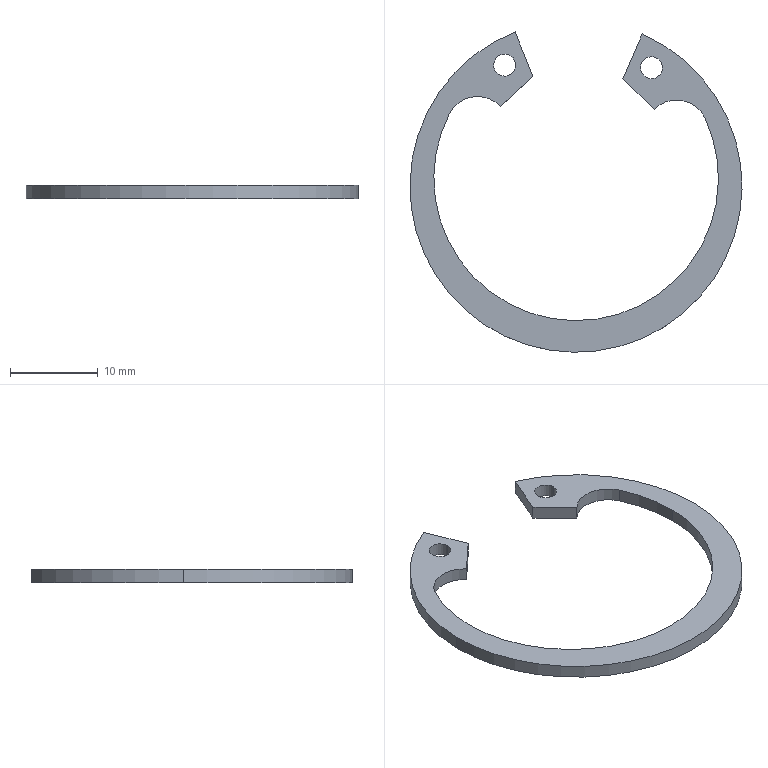Component | SolidWorks | HopperAssembly-1_20211103-210426-70669.STEP-1_-_-_-1.STEP-1_GB893_2-86_B_35.STEP-1 | 1 solid | 18 faces | box 37.8 x 36.49 x 1.5 mm | volume 478 mm3 | cylinder 12 | plane 6 | commonest cylinder face diameters 2.5 x4 32.4 x3 37.8 x3 7.2 x2
STEP:
#1=CARTESIAN_POINT('',(-115.828,33.727,-14.858));
#2=VERTEX_POINT('',#1);
#3=CARTESIAN_POINT('',(-115.927,33.729,-14.858));
#4=VERTEX_POINT('',#3);
#5=CARTESIAN_POINT('',(-115.877,33.728,-14.858));
#6=DIRECTION('',(-0.,-0.,1.));
#7=DIRECTION('',(-0.9998,0.01747,0.));
#8=AXIS2_PLACEMENT_3D('',#5,#6,#7);
#9=CIRCLE('',#8,0.04921);
#10=EDGE_CURVE('',#2,#4,#9,.T.);
#11=ORIENTED_EDGE('',*,*,#10,.T.);
#12=CARTESIAN_POINT('',(-115.877,33.728,-14.858));
#13=DIRECTION('',(-0.,-0.,1.));
#14=DIRECTION('',(-0.9998,0.01747,0.));
#15=AXIS2_PLACEMENT_3D('',#12,#13,#14);
#16=CIRCLE('',#15,0.04921);
#17=EDGE_CURVE('',#4,#2,#16,.T.);
#18=ORIENTED_EDGE('',*,*,#17,.T.);
#19=EDGE_LOOP('',(#11,#18));
#20=FACE_BOUND('',#19,.T.);
#21=CARTESIAN_POINT('',(-116.486,33.738,-14.858));
#22=VERTEX_POINT('',#21);
#23=CARTESIAN_POINT('',(-116.585,33.74,-14.858));
#24=VERTEX_POINT('',#23);
#25=CARTESIAN_POINT('',(-116.535,33.739,-14.858));
#26=DIRECTION('',(-0.,-0.,1.));
#27=DIRECTION('',(0.9998,-0.01747,0.));
#28=AXIS2_PLACEMENT_3D('',#25,#26,#27);
#29=CIRCLE('',#28,0.04921);
#30=EDGE_CURVE('',#22,#24,#29,.T.);
#31=ORIENTED_EDGE('',*,*,#30,.T.);
#32=CARTESIAN_POINT('',(-116.535,33.739,-14.858));
#33=DIRECTION('',(-0.,-0.,1.));
#34=DIRECTION('',(0.9998,-0.01747,0.));
#35=AXIS2_PLACEMENT_3D('',#32,#33,#34);
#36=CIRCLE('',#35,0.04921);
#37=EDGE_CURVE('',#24,#22,#36,.T.);
#38=ORIENTED_EDGE('',*,*,#37,.T.);
#39=EDGE_LOOP('',(#31,#38));
#40=FACE_BOUND('',#39,.T.);
#41=CARTESIAN_POINT('',(-116.489,33.889,-14.858));
#42=VERTEX_POINT('',#41);
#43=CARTESIAN_POINT('',(-116.96,33.209,-14.858));
#44=VERTEX_POINT('',#43);
#45=CARTESIAN_POINT('',(-116.216,33.196,-14.858));
#46=DIRECTION('',(-0.,-0.,1.));
#47=DIRECTION('',(-0.9998,0.01747,0.));
#48=AXIS2_PLACEMENT_3D('',#45,#46,#47);
#49=CIRCLE('',#48,0.7441);
#50=EDGE_CURVE('',#42,#44,#49,.T.);
#51=ORIENTED_EDGE('',*,*,#50,.F.);
#52=CARTESIAN_POINT('',(-116.409,33.687,-14.858));
#53=VERTEX_POINT('',#52);
#54=CARTESIAN_POINT('',(-116.409,33.687,-14.858));
#55=DIRECTION('',(-0.3665,0.9304,0.));
#56=VECTOR('',#55,39.37);
#57=LINE('',#54,#56);
#58=EDGE_CURVE('',#53,#42,#57,.T.);
#59=ORIENTED_EDGE('',*,*,#58,.F.);
#60=CARTESIAN_POINT('',(-116.553,33.553,-14.858));
#61=VERTEX_POINT('',#60);
#62=CARTESIAN_POINT('',(-116.553,33.553,-14.858));
#63=DIRECTION('',(0.7328,0.6804,0.));
#64=VECTOR('',#63,39.37);
#65=LINE('',#62,#64);
#66=EDGE_CURVE('',#61,#53,#65,.T.);
#67=ORIENTED_EDGE('',*,*,#66,.F.);
#68=CARTESIAN_POINT('',(-116.784,33.521,-14.858));
#69=VERTEX_POINT('',#68);
#70=CARTESIAN_POINT('',(-116.657,33.457,-14.858));
#71=DIRECTION('',(0.,0.,-1.));
#72=DIRECTION('',(0.9998,-0.01747,0.));
#73=AXIS2_PLACEMENT_3D('',#70,#71,#72);
#74=CIRCLE('',#73,0.1417);
#75=EDGE_CURVE('',#69,#61,#74,.T.);
#76=ORIENTED_EDGE('',*,*,#75,.F.);
#77=CARTESIAN_POINT('',(-116.853,33.243,-14.858));
#78=VERTEX_POINT('',#77);
#79=CARTESIAN_POINT('',(-116.215,33.232,-14.858));
#80=DIRECTION('',(0.,0.,-1.));
#81=DIRECTION('',(-0.9998,0.01747,0.));
#82=AXIS2_PLACEMENT_3D('',#79,#80,#81);
#83=CIRCLE('',#82,0.6378);
#84=EDGE_CURVE('',#78,#69,#83,.T.);
#85=ORIENTED_EDGE('',*,*,#84,.F.);
#86=CARTESIAN_POINT('',(-115.578,33.221,-14.858));
#87=VERTEX_POINT('',#86);
#88=CARTESIAN_POINT('',(-116.215,33.232,-14.858));
#89=DIRECTION('',(0.,0.,-1.));
#90=DIRECTION('',(-0.9998,0.01747,0.));
#91=AXIS2_PLACEMENT_3D('',#88,#89,#90);
#92=CIRCLE('',#91,0.6378);
#93=EDGE_CURVE('',#87,#78,#92,.T.);
#94=ORIENTED_EDGE('',*,*,#93,.F.);
#95=CARTESIAN_POINT('',(-115.637,33.501,-14.858));
#96=VERTEX_POINT('',#95);
#97=CARTESIAN_POINT('',(-116.215,33.232,-14.858));
#98=DIRECTION('',(0.,0.,-1.));
#99=DIRECTION('',(-0.9998,0.01747,0.));
#100=AXIS2_PLACEMENT_3D('',#97,#98,#99);
#101=CIRCLE('',#100,0.6378);
#102=EDGE_CURVE('',#96,#87,#101,.T.);
#103=ORIENTED_EDGE('',*,*,#102,.F.);
#104=CARTESIAN_POINT('',(-115.866,33.541,-14.858));
#105=VERTEX_POINT('',#104);
#106=CARTESIAN_POINT('',(-115.766,33.441,-14.858));
#107=DIRECTION('',(0.,0.,-1.));
#108=DIRECTION('',(-0.9998,0.01747,0.));
#109=AXIS2_PLACEMENT_3D('',#106,#107,#108);
#110=CIRCLE('',#109,0.1417);
#111=EDGE_CURVE('',#105,#96,#110,.T.);
#112=ORIENTED_EDGE('',*,*,#111,.F.);
#113=CARTESIAN_POINT('',(-116.005,33.68,-14.858));
#114=VERTEX_POINT('',#113);
#115=CARTESIAN_POINT('',(-115.866,33.541,-14.858));
#116=DIRECTION('',(0.7086,-0.7056,-0.));
#117=VECTOR('',#116,39.37);
#118=LINE('',#115,#117);
#119=EDGE_CURVE('',#114,#105,#118,.T.);
#120=ORIENTED_EDGE('',*,*,#119,.F.);
#121=CARTESIAN_POINT('',(-115.919,33.879,-14.858));
#122=VERTEX_POINT('',#121);
#123=CARTESIAN_POINT('',(-116.005,33.68,-14.858));
#124=DIRECTION('',(-0.3988,-0.9171,-0.));
#125=VECTOR('',#124,39.37);
#126=LINE('',#123,#125);
#127=EDGE_CURVE('',#122,#114,#126,.T.);
#128=ORIENTED_EDGE('',*,*,#127,.F.);
#129=CARTESIAN_POINT('',(-115.472,33.183,-14.858));
#130=VERTEX_POINT('',#129);
#131=CARTESIAN_POINT('',(-116.216,33.196,-14.858));
#132=DIRECTION('',(-0.,-0.,1.));
#133=DIRECTION('',(-0.9998,0.01747,0.));
#134=AXIS2_PLACEMENT_3D('',#131,#132,#133);
#135=CIRCLE('',#134,0.7441);
#136=EDGE_CURVE('',#130,#122,#135,.T.);
#137=ORIENTED_EDGE('',*,*,#136,.F.);
#138=CARTESIAN_POINT('',(-116.216,33.196,-14.858));
#139=DIRECTION('',(-0.,-0.,1.));
#140=DIRECTION('',(-0.9998,0.01747,0.));
#141=AXIS2_PLACEMENT_3D('',#138,#139,#140);
#142=CIRCLE('',#141,0.7441);
#143=EDGE_CURVE('',#44,#130,#142,.T.);
#144=ORIENTED_EDGE('',*,*,#143,.F.);
#145=EDGE_LOOP('',(#51,#59,#67,#76,#85,#94,#103,#112,#120,#128,#137,#144));
#146=FACE_OUTER_BOUND('',#145,.T.);
#147=CARTESIAN_POINT('',(-116.216,33.196,-14.858));
#148=DIRECTION('',(-0.,-0.,1.));
#149=DIRECTION('',(-0.9998,0.01747,-0.));
#150=AXIS2_PLACEMENT_3D('',#147,#148,#149);
#151=PLANE('',#150);
#152=ADVANCED_FACE('',(#20,#40,#146),#151,.F.);
#153=CARTESIAN_POINT('',(-116.585,33.74,-14.799));
#154=VERTEX_POINT('',#153);
#155=CARTESIAN_POINT('',(-116.585,33.74,-14.799));
#156=DIRECTION('',(0.,0.,-1.));
#157=VECTOR('',#156,39.37);
#158=LINE('',#155,#157);
#159=EDGE_CURVE('',#154,#24,#158,.T.);
#160=ORIENTED_EDGE('',*,*,#159,.F.);
#161=CARTESIAN_POINT('',(-116.486,33.738,-14.799));
#162=VERTEX_POINT('',#161);
#163=CARTESIAN_POINT('',(-116.535,33.739,-14.799));
#164=DIRECTION('',(-0.,-0.,1.));
#165=DIRECTION('',(0.9998,-0.01747,0.));
#166=AXIS2_PLACEMENT_3D('',#163,#164,#165);
#167=CIRCLE('',#166,0.04921);
#168=EDGE_CURVE('',#154,#162,#167,.T.);
#169=ORIENTED_EDGE('',*,*,#168,.T.);
#170=CARTESIAN_POINT('',(-116.486,33.738,-14.799));
#171=DIRECTION('',(0.,0.,-1.));
#172=VECTOR('',#171,39.37);
#173=LINE('',#170,#172);
#174=EDGE_CURVE('',#162,#22,#173,.T.);
#175=ORIENTED_EDGE('',*,*,#174,.T.);
#176=ORIENTED_EDGE('',*,*,#37,.F.);
#177=EDGE_LOOP('',(#160,#169,#175,#176));
#178=FACE_OUTER_BOUND('',#177,.T.);
#179=CARTESIAN_POINT('',(-116.535,33.739,-14.799));
#180=DIRECTION('',(0.,0.,-1.));
#181=DIRECTION('',(0.9998,-0.01747,0.));
#182=AXIS2_PLACEMENT_3D('',#179,#180,#181);
#183=CYLINDRICAL_SURFACE('',#182,0.04921);
#184=ADVANCED_FACE('',(#178),#183,.F.);
#185=CARTESIAN_POINT('',(-115.927,33.729,-14.799));
#186=VERTEX_POINT('',#185);
#187=CARTESIAN_POINT('',(-115.927,33.729,-14.799));
#188=DIRECTION('',(0.,0.,-1.));
#189=VECTOR('',#188,39.37);
#190=LINE('',#187,#189);
#191=EDGE_CURVE('',#186,#4,#190,.T.);
#192=ORIENTED_EDGE('',*,*,#191,.F.);
#193=CARTESIAN_POINT('',(-115.828,33.727,-14.799));
#194=VERTEX_POINT('',#193);
#195=CARTESIAN_POINT('',(-115.877,33.728,-14.799));
#196=DIRECTION('',(-0.,-0.,1.));
#197=DIRECTION('',(-0.9998,0.01747,0.));
#198=AXIS2_PLACEMENT_3D('',#195,#196,#197);
#199=CIRCLE('',#198,0.04921);
#200=EDGE_CURVE('',#186,#194,#199,.T.);
#201=ORIENTED_EDGE('',*,*,#200,.T.);
#202=CARTESIAN_POINT('',(-115.828,33.727,-14.799));
#203=DIRECTION('',(0.,0.,-1.));
#204=VECTOR('',#203,39.37);
#205=LINE('',#202,#204);
#206=EDGE_CURVE('',#194,#2,#205,.T.);
#207=ORIENTED_EDGE('',*,*,#206,.T.);
#208=ORIENTED_EDGE('',*,*,#17,.F.);
#209=EDGE_LOOP('',(#192,#201,#207,#208));
#210=FACE_OUTER_BOUND('',#209,.T.);
#211=CARTESIAN_POINT('',(-115.877,33.728,-14.799));
#212=DIRECTION('',(0.,0.,-1.));
#213=DIRECTION('',(0.9998,-0.01747,0.));
#214=AXIS2_PLACEMENT_3D('',#211,#212,#213);
#215=CYLINDRICAL_SURFACE('',#214,0.04921);
#216=ADVANCED_FACE('',(#210),#215,.F.);
#217=CARTESIAN_POINT('',(-116.409,33.687,-14.799));
#218=VERTEX_POINT('',#217);
#219=CARTESIAN_POINT('',(-116.409,33.687,-14.799));
#220=DIRECTION('',(0.,0.,-1.));
#221=VECTOR('',#220,39.37);
#222=LINE('',#219,#221);
#223=EDGE_CURVE('',#218,#53,#222,.T.);
#224=ORIENTED_EDGE('',*,*,#223,.T.);
#225=ORIENTED_EDGE('',*,*,#58,.T.);
#226=CARTESIAN_POINT('',(-116.489,33.889,-14.799));
#227=VERTEX_POINT('',#226);
#228=CARTESIAN_POINT('',(-116.489,33.889,-14.799));
#229=DIRECTION('',(0.,0.,-1.));
#230=VECTOR('',#229,39.37);
#231=LINE('',#228,#230);
#232=EDGE_CURVE('',#227,#42,#231,.T.);
#233=ORIENTED_EDGE('',*,*,#232,.F.);
#234=CARTESIAN_POINT('',(-116.409,33.687,-14.799));
#235=DIRECTION('',(-0.3665,0.9304,0.));
#236=VECTOR('',#235,39.37);
#237=LINE('',#234,#236);
#238=EDGE_CURVE('',#218,#227,#237,.T.);
#239=ORIENTED_EDGE('',*,*,#238,.F.);
#240=EDGE_LOOP('',(#224,#225,#233,#239));
#241=FACE_OUTER_BOUND('',#240,.T.);
#242=CARTESIAN_POINT('',(-116.409,33.687,-14.799));
#243=DIRECTION('',(-0.9304,-0.3665,-0.));
#244=DIRECTION('',(0.,0.,-1.));
#245=AXIS2_PLACEMENT_3D('',#242,#243,#244);
#246=PLANE('',#245);
#247=ADVANCED_FACE('',(#241),#246,.F.);
#248=CARTESIAN_POINT('',(-116.553,33.553,-14.799));
#249=VERTEX_POINT('',#248);
#250=CARTESIAN_POINT('',(-116.553,33.553,-14.799));
#251=DIRECTION('',(0.,0.,-1.));
#252=VECTOR('',#251,39.37);
#253=LINE('',#250,#252);
#254=EDGE_CURVE('',#249,#61,#253,.T.);
#255=ORIENTED_EDGE('',*,*,#254,.T.);
#256=ORIENTED_EDGE('',*,*,#66,.T.);
#257=ORIENTED_EDGE('',*,*,#223,.F.);
#258=CARTESIAN_POINT('',(-116.553,33.553,-14.799));
#259=DIRECTION('',(0.7328,0.6804,0.));
#260=VECTOR('',#259,39.37);
#261=LINE('',#258,#260);
#262=EDGE_CURVE('',#249,#218,#261,.T.);
#263=ORIENTED_EDGE('',*,*,#262,.F.);
#264=EDGE_LOOP('',(#255,#256,#257,#263));
#265=FACE_OUTER_BOUND('',#264,.T.);
#266=CARTESIAN_POINT('',(-116.553,33.553,-14.799));
#267=DIRECTION('',(-0.6804,0.7328,0.));
#268=DIRECTION('',(0.,0.,-1.));
#269=AXIS2_PLACEMENT_3D('',#266,#267,#268);
#270=PLANE('',#269);
#271=ADVANCED_FACE('',(#265),#270,.F.);
#272=CARTESIAN_POINT('',(-116.784,33.521,-14.799));
#273=VERTEX_POINT('',#272);
#274=CARTESIAN_POINT('',(-116.784,33.521,-14.799));
#275=DIRECTION('',(0.,0.,-1.));
#276=VECTOR('',#275,39.37);
#277=LINE('',#274,#276);
#278=EDGE_CURVE('',#273,#69,#277,.T.);
#279=ORIENTED_EDGE('',*,*,#278,.T.);
#280=ORIENTED_EDGE('',*,*,#75,.T.);
#281=ORIENTED_EDGE('',*,*,#254,.F.);
#282=CARTESIAN_POINT('',(-116.657,33.457,-14.799));
#283=DIRECTION('',(0.,0.,-1.));
#284=DIRECTION('',(0.9998,-0.01747,0.));
#285=AXIS2_PLACEMENT_3D('',#282,#283,#284);
#286=CIRCLE('',#285,0.1417);
#287=EDGE_CURVE('',#273,#249,#286,.T.);
#288=ORIENTED_EDGE('',*,*,#287,.F.);
#289=EDGE_LOOP('',(#279,#280,#281,#288));
#290=FACE_OUTER_BOUND('',#289,.T.);
#291=CARTESIAN_POINT('',(-116.657,33.457,-14.799));
#292=DIRECTION('',(0.,0.,-1.));
#293=DIRECTION('',(0.9998,-0.01747,0.));
#294=AXIS2_PLACEMENT_3D('',#291,#292,#293);
#295=CYLINDRICAL_SURFACE('',#294,0.1417);
#296=ADVANCED_FACE('',(#290),#295,.F.);
#297=CARTESIAN_POINT('',(-115.578,33.221,-14.799));
#298=VERTEX_POINT('',#297);
#299=CARTESIAN_POINT('',(-115.578,33.221,-14.799));
#300=DIRECTION('',(0.,0.,-1.));
#301=VECTOR('',#300,39.37);
#302=LINE('',#299,#301);
#303=EDGE_CURVE('',#298,#87,#302,.T.);
#304=ORIENTED_EDGE('',*,*,#303,.F.);
#305=CARTESIAN_POINT('',(-115.637,33.501,-14.799));
#306=VERTEX_POINT('',#305);
#307=CARTESIAN_POINT('',(-116.215,33.232,-14.799));
#308=DIRECTION('',(0.,0.,-1.));
#309=DIRECTION('',(-0.9998,0.01747,0.));
#310=AXIS2_PLACEMENT_3D('',#307,#308,#309);
#311=CIRCLE('',#310,0.6378);
#312=EDGE_CURVE('',#306,#298,#311,.T.);
#313=ORIENTED_EDGE('',*,*,#312,.F.);
#314=CARTESIAN_POINT('',(-115.637,33.501,-14.799));
#315=DIRECTION('',(0.,0.,-1.));
#316=VECTOR('',#315,39.37);
#317=LINE('',#314,#316);
#318=EDGE_CURVE('',#306,#96,#317,.T.);
#319=ORIENTED_EDGE('',*,*,#318,.T.);
#320=ORIENTED_EDGE('',*,*,#102,.T.);
#321=EDGE_LOOP('',(#304,#313,#319,#320));
#322=FACE_OUTER_BOUND('',#321,.T.);
#323=CARTESIAN_POINT('',(-116.215,33.232,-14.799));
#324=DIRECTION('',(0.,0.,-1.));
#325=DIRECTION('',(0.9998,-0.01747,0.));
#326=AXIS2_PLACEMENT_3D('',#323,#324,#325);
#327=CYLINDRICAL_SURFACE('',#326,0.6378);
#328=ADVANCED_FACE('',(#322),#327,.F.);
#329=CARTESIAN_POINT('',(-115.866,33.541,-14.799));
#330=VERTEX_POINT('',#329);
#331=CARTESIAN_POINT('',(-115.866,33.541,-14.799));
#332=DIRECTION('',(0.,0.,-1.));
#333=VECTOR('',#332,39.37);
#334=LINE('',#331,#333);
#335=EDGE_CURVE('',#330,#105,#334,.T.);
#336=ORIENTED_EDGE('',*,*,#335,.T.);
#337=ORIENTED_EDGE('',*,*,#111,.T.);
#338=ORIENTED_EDGE('',*,*,#318,.F.);
#339=CARTESIAN_POINT('',(-115.766,33.441,-14.799));
#340=DIRECTION('',(0.,0.,-1.));
#341=DIRECTION('',(-0.9998,0.01747,0.));
#342=AXIS2_PLACEMENT_3D('',#339,#340,#341);
#343=CIRCLE('',#342,0.1417);
#344=EDGE_CURVE('',#330,#306,#343,.T.);
#345=ORIENTED_EDGE('',*,*,#344,.F.);
#346=EDGE_LOOP('',(#336,#337,#338,#345));
#347=FACE_OUTER_BOUND('',#346,.T.);
#348=CARTESIAN_POINT('',(-115.766,33.441,-14.799));
#349=DIRECTION('',(0.,0.,-1.));
#350=DIRECTION('',(0.9998,-0.01747,0.));
#351=AXIS2_PLACEMENT_3D('',#348,#349,#350);
#352=CYLINDRICAL_SURFACE('',#351,0.1417);
#353=ADVANCED_FACE('',(#347),#352,.F.);
#354=CARTESIAN_POINT('',(-116.005,33.68,-14.799));
#355=VERTEX_POINT('',#354);
#356=CARTESIAN_POINT('',(-116.005,33.68,-14.799));
#357=DIRECTION('',(0.,0.,-1.));
#358=VECTOR('',#357,39.37);
#359=LINE('',#356,#358);
#360=EDGE_CURVE('',#355,#114,#359,.T.);
#361=ORIENTED_EDGE('',*,*,#360,.T.);
#362=ORIENTED_EDGE('',*,*,#119,.T.);
#363=ORIENTED_EDGE('',*,*,#335,.F.);
#364=CARTESIAN_POINT('',(-115.866,33.541,-14.799));
#365=DIRECTION('',(0.7086,-0.7056,-0.));
#366=VECTOR('',#365,39.37);
#367=LINE('',#364,#366);
#368=EDGE_CURVE('',#355,#330,#367,.T.);
#369=ORIENTED_EDGE('',*,*,#368,.F.);
#370=EDGE_LOOP('',(#361,#362,#363,#369));
#371=FACE_OUTER_BOUND('',#370,.T.);
#372=CARTESIAN_POINT('',(-115.866,33.541,-14.799));
#373=DIRECTION('',(0.7056,0.7086,0.));
#374=DIRECTION('',(0.7086,-0.7056,-0.));
#375=AXIS2_PLACEMENT_3D('',#372,#373,#374);
#376=PLANE('',#375);
#377=ADVANCED_FACE('',(#371),#376,.F.);
#378=CARTESIAN_POINT('',(-115.919,33.879,-14.799));
#379=VERTEX_POINT('',#378);
#380=CARTESIAN_POINT('',(-115.919,33.879,-14.799));
#381=DIRECTION('',(0.,0.,-1.));
#382=VECTOR('',#381,39.37);
#383=LINE('',#380,#382);
#384=EDGE_CURVE('',#379,#122,#383,.T.);
#385=ORIENTED_EDGE('',*,*,#384,.T.);
#386=ORIENTED_EDGE('',*,*,#127,.T.);
#387=ORIENTED_EDGE('',*,*,#360,.F.);
#388=CARTESIAN_POINT('',(-116.005,33.68,-14.799));
#389=DIRECTION('',(-0.3988,-0.9171,-0.));
#390=VECTOR('',#389,39.37);
#391=LINE('',#388,#390);
#392=EDGE_CURVE('',#379,#355,#391,.T.);
#393=ORIENTED_EDGE('',*,*,#392,.F.);
#394=EDGE_LOOP('',(#385,#386,#387,#393));
#395=FACE_OUTER_BOUND('',#394,.T.);
#396=CARTESIAN_POINT('',(-116.005,33.68,-14.799));
#397=DIRECTION('',(0.9171,-0.3988,0.));
#398=DIRECTION('',(-0.,-0.,1.));
#399=AXIS2_PLACEMENT_3D('',#396,#397,#398);
#400=PLANE('',#399);
#401=ADVANCED_FACE('',(#395),#400,.F.);
#402=CARTESIAN_POINT('',(-116.96,33.209,-14.799));
#403=VERTEX_POINT('',#402);
#404=CARTESIAN_POINT('',(-116.96,33.209,-14.799));
#405=DIRECTION('',(0.,0.,-1.));
#406=VECTOR('',#405,39.37);
#407=LINE('',#404,#406);
#408=EDGE_CURVE('',#403,#44,#407,.T.);
#409=ORIENTED_EDGE('',*,*,#408,.F.);
#410=CARTESIAN_POINT('',(-116.216,33.196,-14.799));
#411=DIRECTION('',(-0.,-0.,1.));
#412=DIRECTION('',(-0.9998,0.01747,0.));
#413=AXIS2_PLACEMENT_3D('',#410,#411,#412);
#414=CIRCLE('',#413,0.7441);
#415=EDGE_CURVE('',#227,#403,#414,.T.);
#416=ORIENTED_EDGE('',*,*,#415,.F.);
#417=ORIENTED_EDGE('',*,*,#232,.T.);
#418=ORIENTED_EDGE('',*,*,#50,.T.);
#419=EDGE_LOOP('',(#409,#416,#417,#418));
#420=FACE_OUTER_BOUND('',#419,.T.);
#421=CARTESIAN_POINT('',(-116.216,33.196,-14.799));
#422=DIRECTION('',(0.,0.,-1.));
#423=DIRECTION('',(0.9998,-0.01747,0.));
#424=AXIS2_PLACEMENT_3D('',#421,#422,#423);
#425=CYLINDRICAL_SURFACE('',#424,0.7441);
#426=ADVANCED_FACE('',(#420),#425,.T.);
#427=CARTESIAN_POINT('',(-116.535,33.739,-14.799));
#428=DIRECTION('',(-0.,-0.,1.));
#429=DIRECTION('',(0.9998,-0.01747,0.));
#430=AXIS2_PLACEMENT_3D('',#427,#428,#429);
#431=CIRCLE('',#430,0.04921);
#432=EDGE_CURVE('',#162,#154,#431,.T.);
#433=ORIENTED_EDGE('',*,*,#432,.F.);
#434=ORIENTED_EDGE('',*,*,#168,.F.);
#435=EDGE_LOOP('',(#433,#434));
#436=FACE_BOUND('',#435,.T.);
#437=CARTESIAN_POINT('',(-115.877,33.728,-14.799));
#438=DIRECTION('',(-0.,-0.,1.));
#439=DIRECTION('',(-0.9998,0.01747,0.));
#440=AXIS2_PLACEMENT_3D('',#437,#438,#439);
#441=CIRCLE('',#440,0.04921);
#442=EDGE_CURVE('',#194,#186,#441,.T.);
#443=ORIENTED_EDGE('',*,*,#442,.F.);
#444=ORIENTED_EDGE('',*,*,#200,.F.);
#445=EDGE_LOOP('',(#443,#444));
#446=FACE_BOUND('',#445,.T.);
#447=ORIENTED_EDGE('',*,*,#415,.T.);
#448=CARTESIAN_POINT('',(-115.472,33.183,-14.799));
#449=VERTEX_POINT('',#448);
#450=CARTESIAN_POINT('',(-116.216,33.196,-14.799));
#451=DIRECTION('',(-0.,-0.,1.));
#452=DIRECTION('',(-0.9998,0.01747,0.));
#453=AXIS2_PLACEMENT_3D('',#450,#451,#452);
#454=CIRCLE('',#453,0.7441);
#455=EDGE_CURVE('',#403,#449,#454,.T.);
#456=ORIENTED_EDGE('',*,*,#455,.T.);
#457=CARTESIAN_POINT('',(-116.216,33.196,-14.799));
#458=DIRECTION('',(-0.,-0.,1.));
#459=DIRECTION('',(-0.9998,0.01747,0.));
#460=AXIS2_PLACEMENT_3D('',#457,#458,#459);
#461=CIRCLE('',#460,0.7441);
#462=EDGE_CURVE('',#449,#379,#461,.T.);
#463=ORIENTED_EDGE('',*,*,#462,.T.);
#464=ORIENTED_EDGE('',*,*,#392,.T.);
#465=ORIENTED_EDGE('',*,*,#368,.T.);
#466=ORIENTED_EDGE('',*,*,#344,.T.);
#467=ORIENTED_EDGE('',*,*,#312,.T.);
#468=CARTESIAN_POINT('',(-116.853,33.243,-14.799));
#469=VERTEX_POINT('',#468);
#470=CARTESIAN_POINT('',(-116.215,33.232,-14.799));
#471=DIRECTION('',(0.,0.,-1.));
#472=DIRECTION('',(-0.9998,0.01747,0.));
#473=AXIS2_PLACEMENT_3D('',#470,#471,#472);
#474=CIRCLE('',#473,0.6378);
#475=EDGE_CURVE('',#298,#469,#474,.T.);
#476=ORIENTED_EDGE('',*,*,#475,.T.);
#477=CARTESIAN_POINT('',(-116.215,33.232,-14.799));
#478=DIRECTION('',(0.,0.,-1.));
#479=DIRECTION('',(-0.9998,0.01747,0.));
#480=AXIS2_PLACEMENT_3D('',#477,#478,#479);
#481=CIRCLE('',#480,0.6378);
#482=EDGE_CURVE('',#469,#273,#481,.T.);
#483=ORIENTED_EDGE('',*,*,#482,.T.);
#484=ORIENTED_EDGE('',*,*,#287,.T.);
#485=ORIENTED_EDGE('',*,*,#262,.T.);
#486=ORIENTED_EDGE('',*,*,#238,.T.);
#487=EDGE_LOOP('',(#447,#456,#463,#464,#465,#466,#467,#476,#483,#484,#485,#486));
#488=FACE_OUTER_BOUND('',#487,.T.);
#489=CARTESIAN_POINT('',(-116.216,33.196,-14.799));
#490=DIRECTION('',(-0.,-0.,1.));
#491=DIRECTION('',(-0.9998,0.01747,-0.));
#492=AXIS2_PLACEMENT_3D('',#489,#490,#491);
#493=PLANE('',#492);
#494=ADVANCED_FACE('',(#436,#446,#488),#493,.T.);
#495=ORIENTED_EDGE('',*,*,#462,.F.);
#496=CARTESIAN_POINT('',(-115.472,33.183,-14.799));
#497=DIRECTION('',(0.,0.,-1.));
#498=VECTOR('',#497,39.37);
#499=LINE('',#496,#498);
#500=EDGE_CURVE('',#449,#130,#499,.T.);
#501=ORIENTED_EDGE('',*,*,#500,.T.);
#502=ORIENTED_EDGE('',*,*,#136,.T.);
#503=ORIENTED_EDGE('',*,*,#384,.F.);
#504=EDGE_LOOP('',(#495,#501,#502,#503));
#505=FACE_OUTER_BOUND('',#504,.T.);
#506=CARTESIAN_POINT('',(-116.216,33.196,-14.799));
#507=DIRECTION('',(0.,0.,-1.));
#508=DIRECTION('',(0.9998,-0.01747,0.));
#509=AXIS2_PLACEMENT_3D('',#506,#507,#508);
#510=CYLINDRICAL_SURFACE('',#509,0.7441);
#511=ADVANCED_FACE('',(#505),#510,.T.);
#512=ORIENTED_EDGE('',*,*,#455,.F.);
#513=ORIENTED_EDGE('',*,*,#408,.T.);
#514=ORIENTED_EDGE('',*,*,#143,.T.);
#515=ORIENTED_EDGE('',*,*,#500,.F.);
#516=EDGE_LOOP('',(#512,#513,#514,#515));
#517=FACE_OUTER_BOUND('',#516,.T.);
#518=CARTESIAN_POINT('',(-116.216,33.196,-14.799));
#519=DIRECTION('',(0.,0.,-1.));
#520=DIRECTION('',(0.9998,-0.01747,0.));
#521=AXIS2_PLACEMENT_3D('',#518,#519,#520);
#522=CYLINDRICAL_SURFACE('',#521,0.7441);
#523=ADVANCED_FACE('',(#517),#522,.T.);
#524=CARTESIAN_POINT('',(-116.853,33.243,-14.799));
#525=DIRECTION('',(0.,0.,-1.));
#526=VECTOR('',#525,39.37);
#527=LINE('',#524,#526);
#528=EDGE_CURVE('',#469,#78,#527,.T.);
#529=ORIENTED_EDGE('',*,*,#528,.F.);
#530=ORIENTED_EDGE('',*,*,#475,.F.);
#531=ORIENTED_EDGE('',*,*,#303,.T.);
#532=ORIENTED_EDGE('',*,*,#93,.T.);
#533=EDGE_LOOP('',(#529,#530,#531,#532));
#534=FACE_OUTER_BOUND('',#533,.T.);
#535=CARTESIAN_POINT('',(-116.215,33.232,-14.799));
#536=DIRECTION('',(0.,0.,-1.));
#537=DIRECTION('',(0.9998,-0.01747,0.));
#538=AXIS2_PLACEMENT_3D('',#535,#536,#537);
#539=CYLINDRICAL_SURFACE('',#538,0.6378);
#540=ADVANCED_FACE('',(#534),#539,.F.);
#541=ORIENTED_EDGE('',*,*,#482,.F.);
#542=ORIENTED_EDGE('',*,*,#528,.T.);
#543=ORIENTED_EDGE('',*,*,#84,.T.);
#544=ORIENTED_EDGE('',*,*,#278,.F.);
#545=EDGE_LOOP('',(#541,#542,#543,#544));
#546=FACE_OUTER_BOUND('',#545,.T.);
#547=CARTESIAN_POINT('',(-116.215,33.232,-14.799));
#548=DIRECTION('',(0.,0.,-1.));
#549=DIRECTION('',(0.9998,-0.01747,0.));
#550=AXIS2_PLACEMENT_3D('',#547,#548,#549);
#551=CYLINDRICAL_SURFACE('',#550,0.6378);
#552=ADVANCED_FACE('',(#546),#551,.F.);
#553=ORIENTED_EDGE('',*,*,#442,.T.);
#554=ORIENTED_EDGE('',*,*,#191,.T.);
#555=ORIENTED_EDGE('',*,*,#10,.F.);
#556=ORIENTED_EDGE('',*,*,#206,.F.);
#557=EDGE_LOOP('',(#553,#554,#555,#556));
#558=FACE_OUTER_BOUND('',#557,.T.);
#559=CARTESIAN_POINT('',(-115.877,33.728,-14.799));
#560=DIRECTION('',(0.,0.,-1.));
#561=DIRECTION('',(0.9998,-0.01747,0.));
#562=AXIS2_PLACEMENT_3D('',#559,#560,#561);
#563=CYLINDRICAL_SURFACE('',#562,0.04921);
#564=ADVANCED_FACE('',(#558),#563,.F.);
#565=ORIENTED_EDGE('',*,*,#432,.T.);
#566=ORIENTED_EDGE('',*,*,#159,.T.);
#567=ORIENTED_EDGE('',*,*,#30,.F.);
#568=ORIENTED_EDGE('',*,*,#174,.F.);
#569=EDGE_LOOP('',(#565,#566,#567,#568));
#570=FACE_OUTER_BOUND('',#569,.T.);
#571=CARTESIAN_POINT('',(-116.535,33.739,-14.799));
#572=DIRECTION('',(0.,0.,-1.));
#573=DIRECTION('',(0.9998,-0.01747,0.));
#574=AXIS2_PLACEMENT_3D('',#571,#572,#573);
#575=CYLINDRICAL_SURFACE('',#574,0.04921);
#576=ADVANCED_FACE('',(#570),#575,.F.);
#577=CLOSED_SHELL('',(#152,#184,#216,#247,#271,#296,#328,#353,#377,#401,#426,#494,#511,#523,#540,#552,#564,#576));
#578=MANIFOLD_SOLID_BREP('',#577);
#579=CARTESIAN_POINT('',(0.,0.,0.));
#580=DIRECTION('',(0.,0.,1.));
#581=DIRECTION('',(1.,0.,0.));
#582=AXIS2_PLACEMENT_3D('',#579,#580,#581);
#583=(LENGTH_UNIT()NAMED_UNIT(*)SI_UNIT($,.METRE.));
#584=LENGTH_MEASURE_WITH_UNIT(LENGTH_MEASURE(0.0254),#583);
#585=DIMENSIONAL_EXPONENTS(1.,0.,0.,0.,0.,0.,0.);
#586=(CONVERSION_BASED_UNIT('',#584)LENGTH_UNIT()NAMED_UNIT(#585));
#587=UNCERTAINTY_MEASURE_WITH_UNIT(LENGTH_MEASURE(0.00001),#586,'','');
#588=(NAMED_UNIT(*)PLANE_ANGLE_UNIT()SI_UNIT($,.RADIAN.));
#589=(NAMED_UNIT(*)SI_UNIT($,.STERADIAN.)SOLID_ANGLE_UNIT());
#590=(GEOMETRIC_REPRESENTATION_CONTEXT(3)GLOBAL_UNCERTAINTY_ASSIGNED_CONTEXT((#587))GLOBAL_UNIT_ASSIGNED_CONTEXT((#586,#588,#589))REPRESENTATION_CONTEXT('',''));
#591=ADVANCED_BREP_SHAPE_REPRESENTATION('',(#578,#582),#590);
#592=COLOUR_RGB('',0.7922,0.8196,0.9333);
#593=FILL_AREA_STYLE_COLOUR('',#592);
#594=FILL_AREA_STYLE('',(#593));
#595=SURFACE_STYLE_FILL_AREA(#594);
#596=SURFACE_SIDE_STYLE('',(#595));
#597=SURFACE_STYLE_USAGE(.BOTH.,#596);
#598=PRESENTATION_STYLE_ASSIGNMENT((#597));
#599=STYLED_ITEM('',(#598),#578);
#600=PRESENTATION_LAYER_ASSIGNMENT('','',(#599));
#601=(LENGTH_UNIT()NAMED_UNIT(*)SI_UNIT($,.METRE.));
#602=LENGTH_MEASURE_WITH_UNIT(LENGTH_MEASURE(0.0254),#601);
#603=DIMENSIONAL_EXPONENTS(1.,0.,0.,0.,0.,0.,0.);
#604=(CONVERSION_BASED_UNIT('',#602)LENGTH_UNIT()NAMED_UNIT(#603));
#605=UNCERTAINTY_MEASURE_WITH_UNIT(LENGTH_MEASURE(0.00001),#604,'','');
#606=(NAMED_UNIT(*)PLANE_ANGLE_UNIT()SI_UNIT($,.RADIAN.));
#607=(NAMED_UNIT(*)SI_UNIT($,.STERADIAN.)SOLID_ANGLE_UNIT());
#608=(GEOMETRIC_REPRESENTATION_CONTEXT(3)GLOBAL_UNCERTAINTY_ASSIGNED_CONTEXT((#605))GLOBAL_UNIT_ASSIGNED_CONTEXT((#604,#606,#607))REPRESENTATION_CONTEXT('',''));
#609=MECHANICAL_DESIGN_GEOMETRIC_PRESENTATION_REPRESENTATION('',(#599),#608);